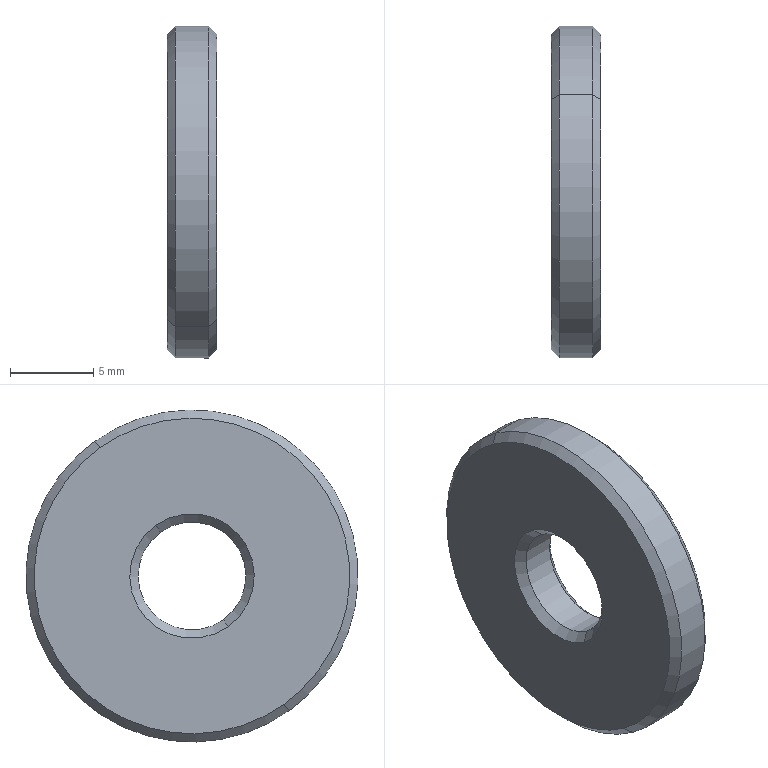Component | SolidWorks | CCD12DriveWheelRetainingRing-2 | 1 solid | 14 faces | box 3 x 20 x 20 mm | volume 822 mm3 | cone 8 | cylinder 4 | plane 2 | commonest cylinder face diameters 6.5 x2 20 x2
build123d program:
from build123d import *

# Parameters (mm, degrees)
SKETCH1_R           = 10
BOSS_EXTRUDE1_DEPTH = 3
SKETCH2_R           = 3.25
CUT_EXTRUDE1_DEPTH  = 15.457
CHAMFER1_SIZE       = 0.5


with BuildPart() as part:
    # Sketch1 → Boss-Extrude1 (new body)
    with BuildSketch(Plane.XY):
        Circle(SKETCH1_R)
    extrude(amount=BOSS_EXTRUDE1_DEPTH)

    # Sketch2 → Cut-Extrude1 (cut, through all)
    with BuildSketch(Plane.XY.offset(3)):
        Circle(SKETCH2_R)
    extrude(amount=-CUT_EXTRUDE1_DEPTH, mode=Mode.SUBTRACT)

    # Chamfer1
    chamfer1_edges = [part.edges().sort_by_distance(p)[0] for p in [
        (-3.25, 0, 0),
        (-3.25, 0, 3),
        (-10, 0, 0),
        (-10, 0, 3),
    ]]
    chamfer(chamfer1_edges, length=CHAMFER1_SIZE)


solid = part.part

# Placed as in the assembly
solid = solid.moved(Location((109.879, 107.251, -99), (0, 90, 0)))
STEP:
#1=CARTESIAN_POINT('',(4.326,4.441,-3.594));
#2=VERTEX_POINT('',#1);
#3=CARTESIAN_POINT('',(4.326,4.004,-4.201));
#4=VERTEX_POINT('',#3);
#5=CARTESIAN_POINT('',(4.326,4.222,-3.898));
#6=DIRECTION('',(-1.,0.,0.));
#7=DIRECTION('',(0.,0.5843,0.8116));
#8=AXIS2_PLACEMENT_3D('',#5,#6,#7);
#9=CIRCLE('',#8,0.374);
#10=EDGE_CURVE('',#2,#4,#9,.T.);
#11=ORIENTED_EDGE('',*,*,#10,.F.);
#12=CARTESIAN_POINT('',(4.346,4.453,-3.578));
#13=VERTEX_POINT('',#12);
#14=CARTESIAN_POINT('',(4.326,4.441,-3.594));
#15=DIRECTION('',(0.7071,0.4131,0.5739));
#16=VECTOR('',#15,39.37);
#17=LINE('',#14,#16);
#18=EDGE_CURVE('',#2,#13,#17,.T.);
#19=ORIENTED_EDGE('',*,*,#18,.T.);
#20=CARTESIAN_POINT('',(4.346,3.992,-4.217));
#21=VERTEX_POINT('',#20);
#22=CARTESIAN_POINT('',(4.346,4.222,-3.898));
#23=DIRECTION('',(1.,-0.,-0.));
#24=DIRECTION('',(0.,0.5843,0.8116));
#25=AXIS2_PLACEMENT_3D('',#22,#23,#24);
#26=CIRCLE('',#25,0.3937);
#27=EDGE_CURVE('',#21,#13,#26,.T.);
#28=ORIENTED_EDGE('',*,*,#27,.F.);
#29=CARTESIAN_POINT('',(4.326,4.004,-4.201));
#30=DIRECTION('',(0.7071,-0.4131,-0.5739));
#31=VECTOR('',#30,39.37);
#32=LINE('',#29,#31);
#33=EDGE_CURVE('',#4,#21,#32,.T.);
#34=ORIENTED_EDGE('',*,*,#33,.F.);
#35=EDGE_LOOP('',(#11,#19,#28,#34));
#36=FACE_OUTER_BOUND('',#35,.T.);
#37=CARTESIAN_POINT('',(4.326,4.222,-3.898));
#38=DIRECTION('',(1.,-0.,-0.));
#39=DIRECTION('',(-0.,-0.5843,-0.8116));
#40=AXIS2_PLACEMENT_3D('',#37,#38,#39);
#41=CONICAL_SURFACE('',#40,0.374,0.7854);
#42=ADVANCED_FACE('',(#36),#41,.T.);
#43=CARTESIAN_POINT('',(4.444,4.004,-4.201));
#44=VERTEX_POINT('',#43);
#45=CARTESIAN_POINT('',(4.444,4.441,-3.594));
#46=VERTEX_POINT('',#45);
#47=CARTESIAN_POINT('',(4.444,4.222,-3.898));
#48=DIRECTION('',(1.,-0.,-0.));
#49=DIRECTION('',(0.,0.5843,0.8116));
#50=AXIS2_PLACEMENT_3D('',#47,#48,#49);
#51=CIRCLE('',#50,0.374);
#52=EDGE_CURVE('',#44,#46,#51,.T.);
#53=ORIENTED_EDGE('',*,*,#52,.F.);
#54=CARTESIAN_POINT('',(4.424,3.992,-4.217));
#55=VERTEX_POINT('',#54);
#56=CARTESIAN_POINT('',(4.424,3.992,-4.217));
#57=DIRECTION('',(-0.7071,-0.4131,-0.5739));
#58=VECTOR('',#57,39.37);
#59=LINE('',#56,#58);
#60=EDGE_CURVE('',#44,#55,#59,.T.);
#61=ORIENTED_EDGE('',*,*,#60,.T.);
#62=CARTESIAN_POINT('',(4.424,4.453,-3.578));
#63=VERTEX_POINT('',#62);
#64=CARTESIAN_POINT('',(4.424,4.222,-3.898));
#65=DIRECTION('',(-1.,0.,0.));
#66=DIRECTION('',(0.,0.5843,0.8116));
#67=AXIS2_PLACEMENT_3D('',#64,#65,#66);
#68=CIRCLE('',#67,0.3937);
#69=EDGE_CURVE('',#63,#55,#68,.T.);
#70=ORIENTED_EDGE('',*,*,#69,.F.);
#71=CARTESIAN_POINT('',(4.424,4.453,-3.578));
#72=DIRECTION('',(-0.7071,0.4131,0.5739));
#73=VECTOR('',#72,39.37);
#74=LINE('',#71,#73);
#75=EDGE_CURVE('',#46,#63,#74,.T.);
#76=ORIENTED_EDGE('',*,*,#75,.F.);
#77=EDGE_LOOP('',(#53,#61,#70,#76));
#78=FACE_OUTER_BOUND('',#77,.T.);
#79=CARTESIAN_POINT('',(4.424,4.222,-3.898));
#80=DIRECTION('',(-1.,0.,0.));
#81=DIRECTION('',(0.,0.5843,0.8116));
#82=AXIS2_PLACEMENT_3D('',#79,#80,#81);
#83=CONICAL_SURFACE('',#82,0.3937,0.7854);
#84=ADVANCED_FACE('',(#78),#83,.T.);
#85=CARTESIAN_POINT('',(4.346,4.148,-4.001));
#86=VERTEX_POINT('',#85);
#87=CARTESIAN_POINT('',(4.346,4.297,-3.794));
#88=VERTEX_POINT('',#87);
#89=CARTESIAN_POINT('',(4.346,4.222,-3.898));
#90=DIRECTION('',(-1.,0.,0.));
#91=DIRECTION('',(0.,0.5843,0.8116));
#92=AXIS2_PLACEMENT_3D('',#89,#90,#91);
#93=CIRCLE('',#92,0.128);
#94=EDGE_CURVE('',#86,#88,#93,.T.);
#95=ORIENTED_EDGE('',*,*,#94,.F.);
#96=CARTESIAN_POINT('',(4.326,4.136,-4.017));
#97=VERTEX_POINT('',#96);
#98=CARTESIAN_POINT('',(4.346,4.148,-4.001));
#99=DIRECTION('',(-0.7071,-0.4131,-0.5739));
#100=VECTOR('',#99,39.37);
#101=LINE('',#98,#100);
#102=EDGE_CURVE('',#86,#97,#101,.T.);
#103=ORIENTED_EDGE('',*,*,#102,.T.);
#104=CARTESIAN_POINT('',(4.326,4.309,-3.778));
#105=VERTEX_POINT('',#104);
#106=CARTESIAN_POINT('',(4.326,4.222,-3.898));
#107=DIRECTION('',(1.,-0.,-0.));
#108=DIRECTION('',(0.,0.5843,0.8116));
#109=AXIS2_PLACEMENT_3D('',#106,#107,#108);
#110=CIRCLE('',#109,0.1476);
#111=EDGE_CURVE('',#105,#97,#110,.T.);
#112=ORIENTED_EDGE('',*,*,#111,.F.);
#113=CARTESIAN_POINT('',(4.346,4.297,-3.794));
#114=DIRECTION('',(-0.7071,0.4131,0.5739));
#115=VECTOR('',#114,39.37);
#116=LINE('',#113,#115);
#117=EDGE_CURVE('',#88,#105,#116,.T.);
#118=ORIENTED_EDGE('',*,*,#117,.F.);
#119=EDGE_LOOP('',(#95,#103,#112,#118));
#120=FACE_OUTER_BOUND('',#119,.T.);
#121=CARTESIAN_POINT('',(4.346,4.222,-3.898));
#122=DIRECTION('',(-1.,0.,0.));
#123=DIRECTION('',(0.,0.5843,0.8116));
#124=AXIS2_PLACEMENT_3D('',#121,#122,#123);
#125=CONICAL_SURFACE('',#124,0.128,0.7854);
#126=ADVANCED_FACE('',(#120),#125,.F.);
#127=CARTESIAN_POINT('',(4.424,4.297,-3.794));
#128=VERTEX_POINT('',#127);
#129=CARTESIAN_POINT('',(4.424,4.148,-4.001));
#130=VERTEX_POINT('',#129);
#131=CARTESIAN_POINT('',(4.424,4.222,-3.898));
#132=DIRECTION('',(1.,-0.,-0.));
#133=DIRECTION('',(0.,0.5843,0.8116));
#134=AXIS2_PLACEMENT_3D('',#131,#132,#133);
#135=CIRCLE('',#134,0.128);
#136=EDGE_CURVE('',#128,#130,#135,.T.);
#137=ORIENTED_EDGE('',*,*,#136,.F.);
#138=CARTESIAN_POINT('',(4.444,4.309,-3.778));
#139=VERTEX_POINT('',#138);
#140=CARTESIAN_POINT('',(4.444,4.309,-3.778));
#141=DIRECTION('',(0.7071,0.4131,0.5739));
#142=VECTOR('',#141,39.37);
#143=LINE('',#140,#142);
#144=EDGE_CURVE('',#128,#139,#143,.T.);
#145=ORIENTED_EDGE('',*,*,#144,.T.);
#146=CARTESIAN_POINT('',(4.444,4.136,-4.017));
#147=VERTEX_POINT('',#146);
#148=CARTESIAN_POINT('',(4.444,4.222,-3.898));
#149=DIRECTION('',(-1.,0.,0.));
#150=DIRECTION('',(0.,0.5843,0.8116));
#151=AXIS2_PLACEMENT_3D('',#148,#149,#150);
#152=CIRCLE('',#151,0.1476);
#153=EDGE_CURVE('',#147,#139,#152,.T.);
#154=ORIENTED_EDGE('',*,*,#153,.F.);
#155=CARTESIAN_POINT('',(4.444,4.136,-4.017));
#156=DIRECTION('',(0.7071,-0.4131,-0.5739));
#157=VECTOR('',#156,39.37);
#158=LINE('',#155,#157);
#159=EDGE_CURVE('',#130,#147,#158,.T.);
#160=ORIENTED_EDGE('',*,*,#159,.F.);
#161=EDGE_LOOP('',(#137,#145,#154,#160));
#162=FACE_OUTER_BOUND('',#161,.T.);
#163=CARTESIAN_POINT('',(4.444,4.222,-3.898));
#164=DIRECTION('',(1.,-0.,-0.));
#165=DIRECTION('',(-0.,-0.5843,-0.8116));
#166=AXIS2_PLACEMENT_3D('',#163,#164,#165);
#167=CONICAL_SURFACE('',#166,0.1476,0.7854);
#168=ADVANCED_FACE('',(#162),#167,.F.);
#169=ORIENTED_EDGE('',*,*,#136,.T.);
#170=CARTESIAN_POINT('',(4.444,4.148,-4.001));
#171=DIRECTION('',(-1.,0.,0.));
#172=VECTOR('',#171,39.37);
#173=LINE('',#170,#172);
#174=EDGE_CURVE('',#130,#86,#173,.T.);
#175=ORIENTED_EDGE('',*,*,#174,.T.);
#176=ORIENTED_EDGE('',*,*,#94,.T.);
#177=CARTESIAN_POINT('',(4.444,4.297,-3.794));
#178=DIRECTION('',(-1.,0.,0.));
#179=VECTOR('',#178,39.37);
#180=LINE('',#177,#179);
#181=EDGE_CURVE('',#128,#88,#180,.T.);
#182=ORIENTED_EDGE('',*,*,#181,.F.);
#183=EDGE_LOOP('',(#169,#175,#176,#182));
#184=FACE_OUTER_BOUND('',#183,.T.);
#185=CARTESIAN_POINT('',(4.444,4.222,-3.898));
#186=DIRECTION('',(-1.,0.,0.));
#187=DIRECTION('',(0.,0.5843,0.8116));
#188=AXIS2_PLACEMENT_3D('',#185,#186,#187);
#189=CYLINDRICAL_SURFACE('',#188,0.128);
#190=ADVANCED_FACE('',(#184),#189,.F.);
#191=ORIENTED_EDGE('',*,*,#27,.T.);
#192=CARTESIAN_POINT('',(4.326,4.453,-3.578));
#193=DIRECTION('',(1.,-0.,-0.));
#194=VECTOR('',#193,39.37);
#195=LINE('',#192,#194);
#196=EDGE_CURVE('',#13,#63,#195,.T.);
#197=ORIENTED_EDGE('',*,*,#196,.T.);
#198=ORIENTED_EDGE('',*,*,#69,.T.);
#199=CARTESIAN_POINT('',(4.326,3.992,-4.217));
#200=DIRECTION('',(1.,-0.,-0.));
#201=VECTOR('',#200,39.37);
#202=LINE('',#199,#201);
#203=EDGE_CURVE('',#21,#55,#202,.T.);
#204=ORIENTED_EDGE('',*,*,#203,.F.);
#205=EDGE_LOOP('',(#191,#197,#198,#204));
#206=FACE_OUTER_BOUND('',#205,.T.);
#207=CARTESIAN_POINT('',(4.326,4.222,-3.898));
#208=DIRECTION('',(1.,-0.,-0.));
#209=DIRECTION('',(-0.,-0.5843,-0.8116));
#210=AXIS2_PLACEMENT_3D('',#207,#208,#209);
#211=CYLINDRICAL_SURFACE('',#210,0.3937);
#212=ADVANCED_FACE('',(#206),#211,.T.);
#213=ORIENTED_EDGE('',*,*,#196,.F.);
#214=CARTESIAN_POINT('',(4.346,4.222,-3.898));
#215=DIRECTION('',(1.,-0.,-0.));
#216=DIRECTION('',(0.,0.5843,0.8116));
#217=AXIS2_PLACEMENT_3D('',#214,#215,#216);
#218=CIRCLE('',#217,0.3937);
#219=EDGE_CURVE('',#13,#21,#218,.T.);
#220=ORIENTED_EDGE('',*,*,#219,.T.);
#221=ORIENTED_EDGE('',*,*,#203,.T.);
#222=CARTESIAN_POINT('',(4.424,4.222,-3.898));
#223=DIRECTION('',(-1.,0.,0.));
#224=DIRECTION('',(0.,0.5843,0.8116));
#225=AXIS2_PLACEMENT_3D('',#222,#223,#224);
#226=CIRCLE('',#225,0.3937);
#227=EDGE_CURVE('',#55,#63,#226,.T.);
#228=ORIENTED_EDGE('',*,*,#227,.T.);
#229=EDGE_LOOP('',(#213,#220,#221,#228));
#230=FACE_OUTER_BOUND('',#229,.T.);
#231=CARTESIAN_POINT('',(4.326,4.222,-3.898));
#232=DIRECTION('',(1.,-0.,-0.));
#233=DIRECTION('',(-0.,-0.5843,-0.8116));
#234=AXIS2_PLACEMENT_3D('',#231,#232,#233);
#235=CYLINDRICAL_SURFACE('',#234,0.3937);
#236=ADVANCED_FACE('',(#230),#235,.T.);
#237=ORIENTED_EDGE('',*,*,#111,.T.);
#238=CARTESIAN_POINT('',(4.326,4.222,-3.898));
#239=DIRECTION('',(1.,-0.,-0.));
#240=DIRECTION('',(0.,0.5843,0.8116));
#241=AXIS2_PLACEMENT_3D('',#238,#239,#240);
#242=CIRCLE('',#241,0.1476);
#243=EDGE_CURVE('',#97,#105,#242,.T.);
#244=ORIENTED_EDGE('',*,*,#243,.T.);
#245=EDGE_LOOP('',(#237,#244));
#246=FACE_BOUND('',#245,.T.);
#247=CARTESIAN_POINT('',(4.326,4.222,-3.898));
#248=DIRECTION('',(-1.,0.,0.));
#249=DIRECTION('',(0.,0.5843,0.8116));
#250=AXIS2_PLACEMENT_3D('',#247,#248,#249);
#251=CIRCLE('',#250,0.374);
#252=EDGE_CURVE('',#4,#2,#251,.T.);
#253=ORIENTED_EDGE('',*,*,#252,.T.);
#254=ORIENTED_EDGE('',*,*,#10,.T.);
#255=EDGE_LOOP('',(#253,#254));
#256=FACE_OUTER_BOUND('',#255,.T.);
#257=CARTESIAN_POINT('',(4.326,4.222,-3.898));
#258=DIRECTION('',(-1.,0.,0.));
#259=DIRECTION('',(0.,0.5843,0.8116));
#260=AXIS2_PLACEMENT_3D('',#257,#258,#259);
#261=PLANE('',#260);
#262=ADVANCED_FACE('',(#246,#256),#261,.T.);
#263=ORIENTED_EDGE('',*,*,#153,.T.);
#264=CARTESIAN_POINT('',(4.444,4.222,-3.898));
#265=DIRECTION('',(-1.,0.,0.));
#266=DIRECTION('',(0.,0.5843,0.8116));
#267=AXIS2_PLACEMENT_3D('',#264,#265,#266);
#268=CIRCLE('',#267,0.1476);
#269=EDGE_CURVE('',#139,#147,#268,.T.);
#270=ORIENTED_EDGE('',*,*,#269,.T.);
#271=EDGE_LOOP('',(#263,#270));
#272=FACE_BOUND('',#271,.T.);
#273=CARTESIAN_POINT('',(4.444,4.222,-3.898));
#274=DIRECTION('',(1.,-0.,-0.));
#275=DIRECTION('',(0.,0.5843,0.8116));
#276=AXIS2_PLACEMENT_3D('',#273,#274,#275);
#277=CIRCLE('',#276,0.374);
#278=EDGE_CURVE('',#46,#44,#277,.T.);
#279=ORIENTED_EDGE('',*,*,#278,.T.);
#280=ORIENTED_EDGE('',*,*,#52,.T.);
#281=EDGE_LOOP('',(#279,#280));
#282=FACE_OUTER_BOUND('',#281,.T.);
#283=CARTESIAN_POINT('',(4.444,4.222,-3.898));
#284=DIRECTION('',(-1.,0.,0.));
#285=DIRECTION('',(0.,0.5843,0.8116));
#286=AXIS2_PLACEMENT_3D('',#283,#284,#285);
#287=PLANE('',#286);
#288=ADVANCED_FACE('',(#272,#282),#287,.F.);
#289=ORIENTED_EDGE('',*,*,#174,.F.);
#290=CARTESIAN_POINT('',(4.424,4.222,-3.898));
#291=DIRECTION('',(1.,-0.,-0.));
#292=DIRECTION('',(0.,0.5843,0.8116));
#293=AXIS2_PLACEMENT_3D('',#290,#291,#292);
#294=CIRCLE('',#293,0.128);
#295=EDGE_CURVE('',#130,#128,#294,.T.);
#296=ORIENTED_EDGE('',*,*,#295,.T.);
#297=ORIENTED_EDGE('',*,*,#181,.T.);
#298=CARTESIAN_POINT('',(4.346,4.222,-3.898));
#299=DIRECTION('',(-1.,0.,0.));
#300=DIRECTION('',(0.,0.5843,0.8116));
#301=AXIS2_PLACEMENT_3D('',#298,#299,#300);
#302=CIRCLE('',#301,0.128);
#303=EDGE_CURVE('',#88,#86,#302,.T.);
#304=ORIENTED_EDGE('',*,*,#303,.T.);
#305=EDGE_LOOP('',(#289,#296,#297,#304));
#306=FACE_OUTER_BOUND('',#305,.T.);
#307=CARTESIAN_POINT('',(4.444,4.222,-3.898));
#308=DIRECTION('',(-1.,0.,0.));
#309=DIRECTION('',(0.,0.5843,0.8116));
#310=AXIS2_PLACEMENT_3D('',#307,#308,#309);
#311=CYLINDRICAL_SURFACE('',#310,0.128);
#312=ADVANCED_FACE('',(#306),#311,.F.);
#313=ORIENTED_EDGE('',*,*,#144,.F.);
#314=ORIENTED_EDGE('',*,*,#295,.F.);
#315=ORIENTED_EDGE('',*,*,#159,.T.);
#316=ORIENTED_EDGE('',*,*,#269,.F.);
#317=EDGE_LOOP('',(#313,#314,#315,#316));
#318=FACE_OUTER_BOUND('',#317,.T.);
#319=CARTESIAN_POINT('',(4.444,4.222,-3.898));
#320=DIRECTION('',(1.,-0.,-0.));
#321=DIRECTION('',(-0.,-0.5843,-0.8116));
#322=AXIS2_PLACEMENT_3D('',#319,#320,#321);
#323=CONICAL_SURFACE('',#322,0.1476,0.7854);
#324=ADVANCED_FACE('',(#318),#323,.F.);
#325=ORIENTED_EDGE('',*,*,#102,.F.);
#326=ORIENTED_EDGE('',*,*,#303,.F.);
#327=ORIENTED_EDGE('',*,*,#117,.T.);
#328=ORIENTED_EDGE('',*,*,#243,.F.);
#329=EDGE_LOOP('',(#325,#326,#327,#328));
#330=FACE_OUTER_BOUND('',#329,.T.);
#331=CARTESIAN_POINT('',(4.346,4.222,-3.898));
#332=DIRECTION('',(-1.,0.,0.));
#333=DIRECTION('',(0.,0.5843,0.8116));
#334=AXIS2_PLACEMENT_3D('',#331,#332,#333);
#335=CONICAL_SURFACE('',#334,0.128,0.7854);
#336=ADVANCED_FACE('',(#330),#335,.F.);
#337=ORIENTED_EDGE('',*,*,#60,.F.);
#338=ORIENTED_EDGE('',*,*,#278,.F.);
#339=ORIENTED_EDGE('',*,*,#75,.T.);
#340=ORIENTED_EDGE('',*,*,#227,.F.);
#341=EDGE_LOOP('',(#337,#338,#339,#340));
#342=FACE_OUTER_BOUND('',#341,.T.);
#343=CARTESIAN_POINT('',(4.424,4.222,-3.898));
#344=DIRECTION('',(-1.,0.,0.));
#345=DIRECTION('',(0.,0.5843,0.8116));
#346=AXIS2_PLACEMENT_3D('',#343,#344,#345);
#347=CONICAL_SURFACE('',#346,0.3937,0.7854);
#348=ADVANCED_FACE('',(#342),#347,.T.);
#349=ORIENTED_EDGE('',*,*,#18,.F.);
#350=ORIENTED_EDGE('',*,*,#252,.F.);
#351=ORIENTED_EDGE('',*,*,#33,.T.);
#352=ORIENTED_EDGE('',*,*,#219,.F.);
#353=EDGE_LOOP('',(#349,#350,#351,#352));
#354=FACE_OUTER_BOUND('',#353,.T.);
#355=CARTESIAN_POINT('',(4.326,4.222,-3.898));
#356=DIRECTION('',(1.,-0.,-0.));
#357=DIRECTION('',(-0.,-0.5843,-0.8116));
#358=AXIS2_PLACEMENT_3D('',#355,#356,#357);
#359=CONICAL_SURFACE('',#358,0.374,0.7854);
#360=ADVANCED_FACE('',(#354),#359,.T.);
#361=CLOSED_SHELL('',(#42,#84,#126,#168,#190,#212,#236,#262,#288,#312,#324,#336,#348,#360));
#362=MANIFOLD_SOLID_BREP('',#361);
#363=CARTESIAN_POINT('',(0.,0.,0.));
#364=DIRECTION('',(0.,0.,1.));
#365=DIRECTION('',(1.,0.,0.));
#366=AXIS2_PLACEMENT_3D('',#363,#364,#365);
#367=(LENGTH_UNIT()NAMED_UNIT(*)SI_UNIT($,.METRE.));
#368=LENGTH_MEASURE_WITH_UNIT(LENGTH_MEASURE(0.0254),#367);
#369=DIMENSIONAL_EXPONENTS(1.,0.,0.,0.,0.,0.,0.);
#370=(CONVERSION_BASED_UNIT('',#368)LENGTH_UNIT()NAMED_UNIT(#369));
#371=UNCERTAINTY_MEASURE_WITH_UNIT(LENGTH_MEASURE(0.00001),#370,'','');
#372=(NAMED_UNIT(*)PLANE_ANGLE_UNIT()SI_UNIT($,.RADIAN.));
#373=(NAMED_UNIT(*)SI_UNIT($,.STERADIAN.)SOLID_ANGLE_UNIT());
#374=(GEOMETRIC_REPRESENTATION_CONTEXT(3)GLOBAL_UNCERTAINTY_ASSIGNED_CONTEXT((#371))GLOBAL_UNIT_ASSIGNED_CONTEXT((#370,#372,#373))REPRESENTATION_CONTEXT('',''));
#375=ADVANCED_BREP_SHAPE_REPRESENTATION('',(#362,#366),#374);
#376=COLOUR_RGB('',0.7922,0.8196,0.9333);
#377=FILL_AREA_STYLE_COLOUR('',#376);
#378=FILL_AREA_STYLE('',(#377));
#379=SURFACE_STYLE_FILL_AREA(#378);
#380=SURFACE_SIDE_STYLE('',(#379));
#381=SURFACE_STYLE_USAGE(.BOTH.,#380);
#382=PRESENTATION_STYLE_ASSIGNMENT((#381));
#383=STYLED_ITEM('',(#382),#362);
#384=(LENGTH_UNIT()NAMED_UNIT(*)SI_UNIT($,.METRE.));
#385=LENGTH_MEASURE_WITH_UNIT(LENGTH_MEASURE(0.0254),#384);
#386=DIMENSIONAL_EXPONENTS(1.,0.,0.,0.,0.,0.,0.);
#387=(CONVERSION_BASED_UNIT('',#385)LENGTH_UNIT()NAMED_UNIT(#386));
#388=UNCERTAINTY_MEASURE_WITH_UNIT(LENGTH_MEASURE(0.00001),#387,'','');
#389=(NAMED_UNIT(*)PLANE_ANGLE_UNIT()SI_UNIT($,.RADIAN.));
#390=(NAMED_UNIT(*)SI_UNIT($,.STERADIAN.)SOLID_ANGLE_UNIT());
#391=(GEOMETRIC_REPRESENTATION_CONTEXT(3)GLOBAL_UNCERTAINTY_ASSIGNED_CONTEXT((#388))GLOBAL_UNIT_ASSIGNED_CONTEXT((#387,#389,#390))REPRESENTATION_CONTEXT('',''));
#392=MECHANICAL_DESIGN_GEOMETRIC_PRESENTATION_REPRESENTATION('',(#383),#391);
#393=PRESENTATION_LAYER_ASSIGNMENT('','',(#383));